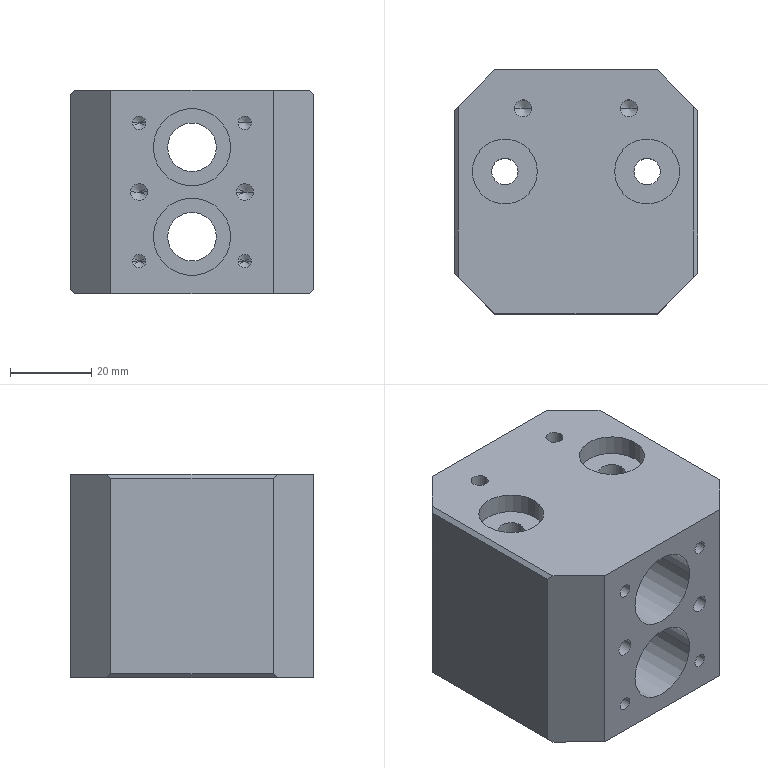Component | SolidWorks | DZ.KX.203-TC1505-30-09-01-05-06-1 | 1 solid | 72 faces | box 60 x 60 x 50 mm | volume 128945 mm3 | cylinder 36 | plane 20 | cone 16 | commonest cylinder face diameters 4.2 x8 3.3 x8 19 x4 12 x4 16 x4 11 x4 6.5 x4 | material 6061 Alloy
build123d program:
from build123d import *

# Parameters (mm, degrees)
SKETCH1_W                                         = 60
SKETCH1_H                                         = 60
BOSS_EXTRUDE1_DEPTH                               = 50
HOLE_SIZE_ACCORDING_TO_HEXAGON_SOCKET_D           = 6.5
HOLE_SIZE_ACCORDING_TO_HEXAGON_SOCKET_CBORE_D     = 11
HOLE_SIZE_ACCORDING_TO_HEXAGON_SOCKET_CBORE_DEPTH = 20
F_16_0_16_DIAMETER_HOLE1_D                        = 16
F_16_0_16_DIAMETER_HOLE1_DEPTH                    = 5
HOLE1_D                                           = 12
HOLE1_CBORE_D                                     = 19
HOLE1_CBORE_DEPTH                                 = 55
M4_TAPPED_HOLE2_D                                 = 3.3
M4_TAPPED_HOLE2_DEPTH                             = 10.1
M4_TAPPED_HOLE2_TIP                               = 0.9914
M5_TAPPED_HOLE2_D                                 = 4.2
M5_TAPPED_HOLE2_DEPTH                             = 15
M5_TAPPED_HOLE2_TIP                               = 1.262
CHAMFER2_SIZE                                     = 1
CHAMFER3_SIZE                                     = 10
M5_TAPPED_HOLE3_D                                 = 4.2
M5_TAPPED_HOLE3_DEPTH                             = 14
M5_TAPPED_HOLE3_TIP                               = 1.262


with BuildPart() as part:
    # Sketch1 → Boss-Extrude1 (new body)
    with BuildSketch(Plane(origin=(0, 0, 0), x_dir=(0, 0, -1), z_dir=(1, 0, 0))):
        Rectangle(SKETCH1_W, SKETCH1_H)
    extrude(amount=BOSS_EXTRUDE1_DEPTH)

    # Hole Size _according to_ Hexagon Socket (through all)
    with Locations(Plane.ZY):
        with Locations((-17.5, 5), (17.5, 5)):
            CounterBoreHole(HOLE_SIZE_ACCORDING_TO_HEXAGON_SOCKET_D / 2, HOLE_SIZE_ACCORDING_TO_HEXAGON_SOCKET_CBORE_D / 2, HOLE_SIZE_ACCORDING_TO_HEXAGON_SOCKET_CBORE_DEPTH)

    # 16.0 _16_ Diameter Hole1
    with Locations(Plane(origin=(50, 0, 0), x_dir=(0, 0, -1), z_dir=(1, 0, 0))):
        with Locations((17.5, 5), (-17.5, 5)):
            Hole(F_16_0_16_DIAMETER_HOLE1_D / 2, depth=F_16_0_16_DIAMETER_HOLE1_DEPTH)

    # Hole1 (through all)
    with Locations(Plane.XZ.offset(30)):
        with Locations((14, 0), (36, 0)):
            CounterBoreHole(HOLE1_D / 2, HOLE1_CBORE_D / 2, HOLE1_CBORE_DEPTH)

    # M4 Tapped Hole2
    with Locations(Plane(origin=(0, -30, 0), x_dir=(-1, 0, 0), z_dir=(0, -1, 0))):
        with Locations((-42, -13), (-8, -13), (-8, 13), (-42, 13)):
            Hole(M4_TAPPED_HOLE2_D / 2, depth=M4_TAPPED_HOLE2_DEPTH)
            with Locations((0, 0, -(M4_TAPPED_HOLE2_DEPTH + M4_TAPPED_HOLE2_TIP / 2))):  # 118° drill point
                Cone(0, M4_TAPPED_HOLE2_D / 2, M4_TAPPED_HOLE2_TIP, mode=Mode.SUBTRACT)

    # M5 Tapped Hole2
    with Locations(Plane(origin=(50, 0, 0), x_dir=(0, 0, -1), z_dir=(1, 0, 0))):
        with Locations((13, 20.5), (-13, 20.5)):
            Hole(M5_TAPPED_HOLE2_D / 2, depth=M5_TAPPED_HOLE2_DEPTH)
            with Locations((0, 0, -(M5_TAPPED_HOLE2_DEPTH + M5_TAPPED_HOLE2_TIP / 2))):  # 118° drill point
                Cone(0, M5_TAPPED_HOLE2_D / 2, M5_TAPPED_HOLE2_TIP, mode=Mode.SUBTRACT)

    # Chamfer2
    chamfer2_edges = [part.edges().sort_by_distance(p)[0] for p in [
        (50, 0, -30),
        (50, 0, 30),
        (0, 0, -30),
        (0, 0, 30),
    ]]
    chamfer(chamfer2_edges, length=CHAMFER2_SIZE)

    # Chamfer3
    chamfer3_edges = [part.edges().sort_by_distance(p)[0] for p in [
        (25, 30, -30),
        (25, 30, 30),
        (25, -30, -30),
        (25, -30, 30),
    ]]
    chamfer(chamfer3_edges, length=CHAMFER3_SIZE)

    # M5 Tapped Hole3
    with Locations(Plane(origin=(0, -30, 0), x_dir=(-1, 0, 0), z_dir=(0, -1, 0))):
        with Locations((-25, 13), (-25, -13)):
            Hole(M5_TAPPED_HOLE3_D / 2, depth=M5_TAPPED_HOLE3_DEPTH)
            with Locations((0, 0, -(M5_TAPPED_HOLE3_DEPTH + M5_TAPPED_HOLE3_TIP / 2))):  # 118° drill point
                Cone(0, M5_TAPPED_HOLE3_D / 2, M5_TAPPED_HOLE3_TIP, mode=Mode.SUBTRACT)


solid = part.part

# Placed as in the assembly
solid = solid.moved(Location((294.5, -615.807, -36.94), (0, -90, 0)))